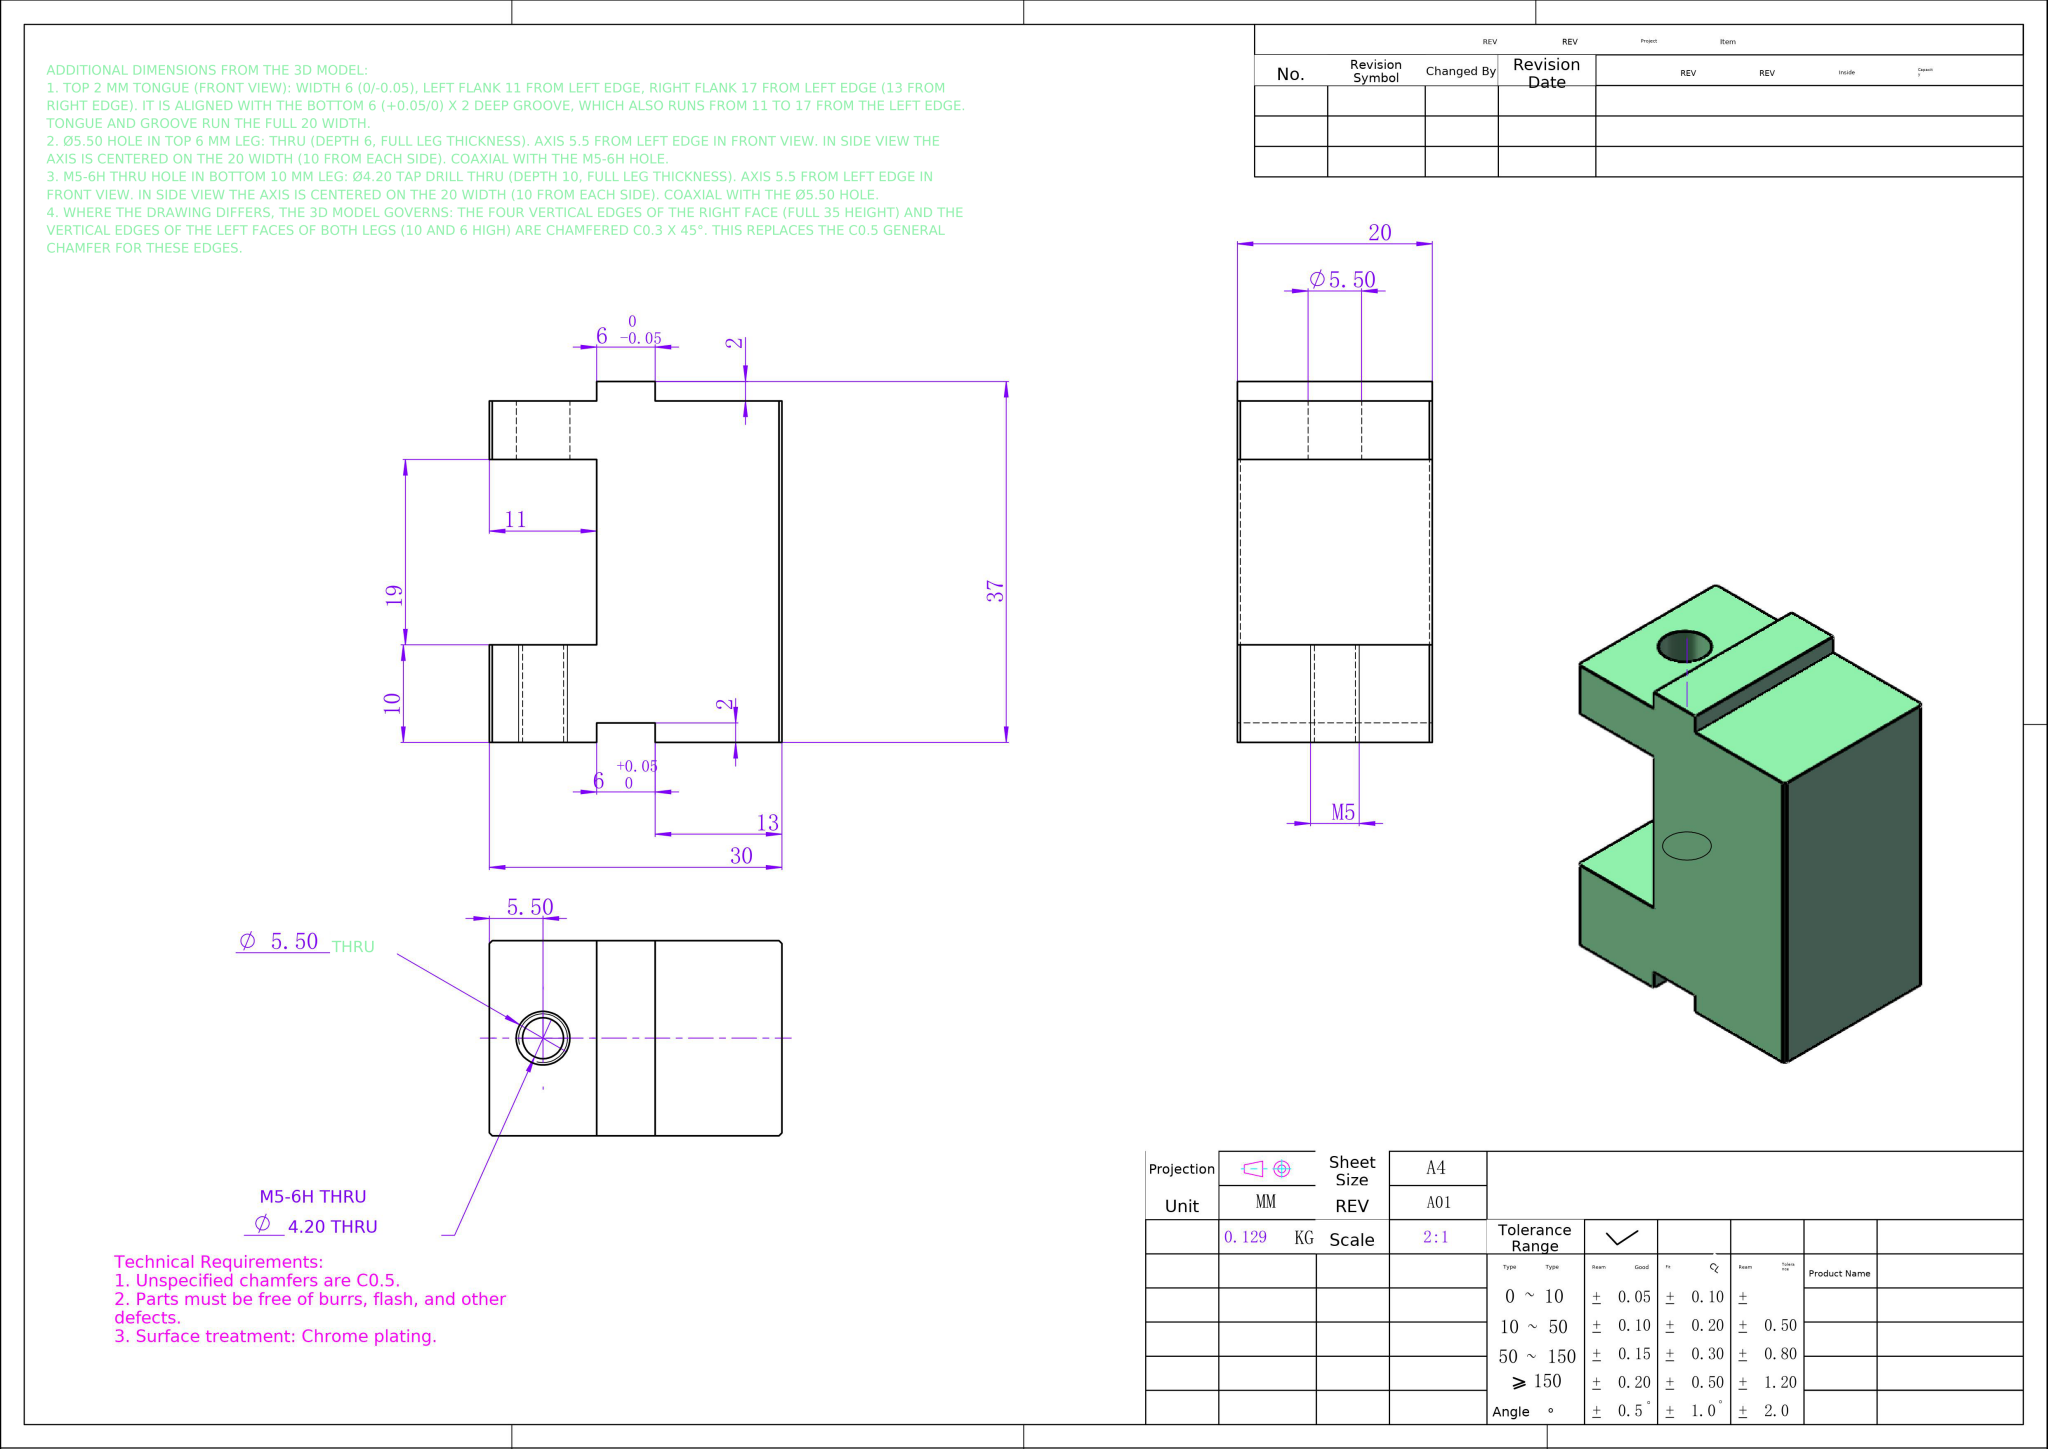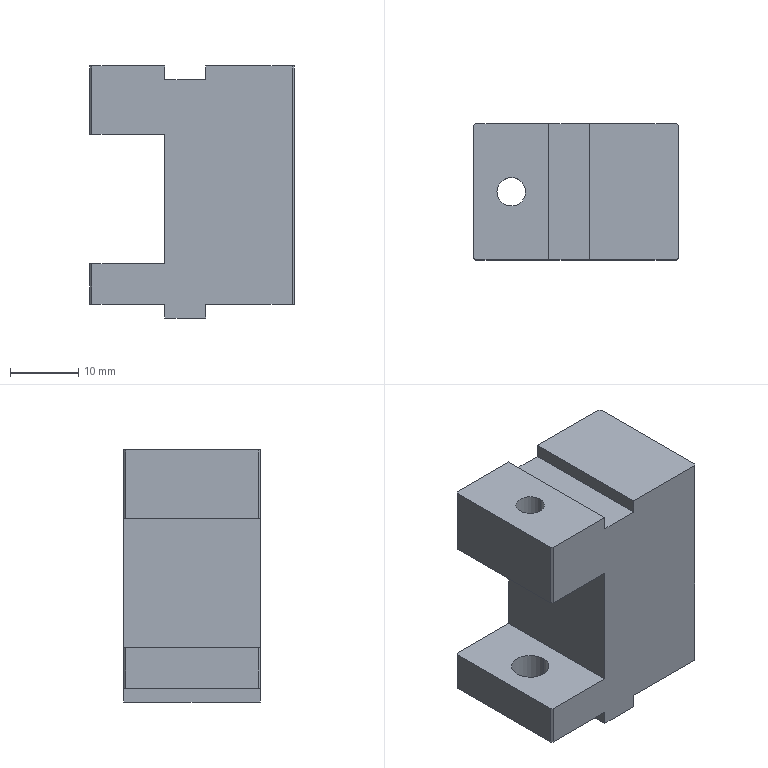Part | NX | mm | 1 solid | 28 faces | box 30 x 20 x 37 mm | volume 16534 mm3 | plane 24 | cylinder 4 | commonest cylinder face diameters 4.2 x2 5.5 x2
STEP:
#1=COLOUR_RGB('',0.5922,1.,0.7098);
#2=FILL_AREA_STYLE_COLOUR('',#1);
#3=FILL_AREA_STYLE('',(#2));
#4=SURFACE_STYLE_FILL_AREA(#3);
#5=SURFACE_SIDE_STYLE('',(#4));
#6=SURFACE_STYLE_USAGE(.BOTH.,#5);
#7=PRESENTATION_STYLE_ASSIGNMENT((#6));
#8=CARTESIAN_POINT('',(-7.4,0.,17.5));
#9=VERTEX_POINT('',#8);
#10=CARTESIAN_POINT('',(-11.6,0.,17.5));
#11=VERTEX_POINT('',#10);
#12=CARTESIAN_POINT('',(-9.5,0.,17.5));
#13=DIRECTION('',(0.,0.,-1.));
#14=DIRECTION('',(-1.,0.,0.));
#15=AXIS2_PLACEMENT_3D('',#12,#13,#14);
#16=CIRCLE('',#15,2.1);
#17=EDGE_CURVE('',#9,#11,#16,.T.);
#18=ORIENTED_EDGE('',*,*,#17,.F.);
#19=CARTESIAN_POINT('',(-7.4,0.,7.5));
#20=VERTEX_POINT('',#19);
#21=CARTESIAN_POINT('',(-7.4,0.,7.5));
#22=DIRECTION('',(0.,0.,-1.));
#23=VECTOR('',#22,1000.);
#24=LINE('',#21,#23);
#25=EDGE_CURVE('',#9,#20,#24,.T.);
#26=ORIENTED_EDGE('',*,*,#25,.T.);
#27=CARTESIAN_POINT('',(-11.6,0.,7.5));
#28=VERTEX_POINT('',#27);
#29=CARTESIAN_POINT('',(-9.5,0.,7.5));
#30=DIRECTION('',(0.,0.,-1.));
#31=DIRECTION('',(-1.,0.,0.));
#32=AXIS2_PLACEMENT_3D('',#29,#30,#31);
#33=CIRCLE('',#32,2.1);
#34=EDGE_CURVE('',#20,#28,#33,.T.);
#35=ORIENTED_EDGE('',*,*,#34,.T.);
#36=CARTESIAN_POINT('',(-11.6,0.,7.5));
#37=DIRECTION('',(0.,0.,-1.));
#38=VECTOR('',#37,1000.);
#39=LINE('',#36,#38);
#40=EDGE_CURVE('',#11,#28,#39,.T.);
#41=ORIENTED_EDGE('',*,*,#40,.F.);
#42=EDGE_LOOP('',(#18,#26,#35,#41));
#43=FACE_OUTER_BOUND('',#42,.T.);
#44=CARTESIAN_POINT('',(-9.5,0.,7.5));
#45=DIRECTION('',(0.,0.,-1.));
#46=DIRECTION('',(-1.,0.,0.));
#47=AXIS2_PLACEMENT_3D('',#44,#45,#46);
#48=CYLINDRICAL_SURFACE('',#47,2.1);
#49=ADVANCED_FACE('',(#43),#48,.F.);
#50=CARTESIAN_POINT('',(-12.25,0.,-11.5));
#51=VERTEX_POINT('',#50);
#52=CARTESIAN_POINT('',(-6.75,0.,-11.5));
#53=VERTEX_POINT('',#52);
#54=CARTESIAN_POINT('',(-9.5,0.,-11.5));
#55=DIRECTION('',(-0.,0.,1.));
#56=DIRECTION('',(-1.,0.,0.));
#57=AXIS2_PLACEMENT_3D('',#54,#55,#56);
#58=CIRCLE('',#57,2.75);
#59=EDGE_CURVE('',#51,#53,#58,.T.);
#60=ORIENTED_EDGE('',*,*,#59,.T.);
#61=CARTESIAN_POINT('',(-6.75,0.,-17.5));
#62=VERTEX_POINT('',#61);
#63=CARTESIAN_POINT('',(-6.75,0.,-17.5));
#64=DIRECTION('',(0.,0.,-1.));
#65=VECTOR('',#64,1000.);
#66=LINE('',#63,#65);
#67=EDGE_CURVE('',#53,#62,#66,.T.);
#68=ORIENTED_EDGE('',*,*,#67,.T.);
#69=CARTESIAN_POINT('',(-12.25,0.,-17.5));
#70=VERTEX_POINT('',#69);
#71=CARTESIAN_POINT('',(-9.5,0.,-17.5));
#72=DIRECTION('',(0.,0.,-1.));
#73=DIRECTION('',(-1.,0.,0.));
#74=AXIS2_PLACEMENT_3D('',#71,#72,#73);
#75=CIRCLE('',#74,2.75);
#76=EDGE_CURVE('',#62,#70,#75,.T.);
#77=ORIENTED_EDGE('',*,*,#76,.T.);
#78=CARTESIAN_POINT('',(-12.25,0.,-17.5));
#79=DIRECTION('',(0.,0.,-1.));
#80=VECTOR('',#79,1000.);
#81=LINE('',#78,#80);
#82=EDGE_CURVE('',#51,#70,#81,.T.);
#83=ORIENTED_EDGE('',*,*,#82,.F.);
#84=EDGE_LOOP('',(#60,#68,#77,#83));
#85=FACE_OUTER_BOUND('',#84,.T.);
#86=CARTESIAN_POINT('',(-9.5,0.,-17.5));
#87=DIRECTION('',(0.,0.,-1.));
#88=DIRECTION('',(-1.,0.,0.));
#89=AXIS2_PLACEMENT_3D('',#86,#87,#88);
#90=CYLINDRICAL_SURFACE('',#89,2.75);
#91=ADVANCED_FACE('',(#85),#90,.F.);
#92=CARTESIAN_POINT('',(-14.7,-10.,7.5));
#93=VERTEX_POINT('',#92);
#94=CARTESIAN_POINT('',(-15.,-9.7,7.5));
#95=VERTEX_POINT('',#94);
#96=CARTESIAN_POINT('',(-14.7,-10.,7.5));
#97=DIRECTION('',(-0.7071,0.7071,-0.));
#98=VECTOR('',#97,1000.);
#99=LINE('',#96,#98);
#100=EDGE_CURVE('',#93,#95,#99,.T.);
#101=ORIENTED_EDGE('',*,*,#100,.T.);
#102=CARTESIAN_POINT('',(-15.,9.7,7.5));
#103=VERTEX_POINT('',#102);
#104=CARTESIAN_POINT('',(-15.,-10.,7.5));
#105=DIRECTION('',(0.,-1.,0.));
#106=VECTOR('',#105,1000.);
#107=LINE('',#104,#106);
#108=EDGE_CURVE('',#103,#95,#107,.T.);
#109=ORIENTED_EDGE('',*,*,#108,.F.);
#110=CARTESIAN_POINT('',(-14.7,10.,7.5));
#111=VERTEX_POINT('',#110);
#112=CARTESIAN_POINT('',(-15.,9.7,7.5));
#113=DIRECTION('',(0.7071,0.7071,0.));
#114=VECTOR('',#113,1000.);
#115=LINE('',#112,#114);
#116=EDGE_CURVE('',#103,#111,#115,.T.);
#117=ORIENTED_EDGE('',*,*,#116,.T.);
#118=CARTESIAN_POINT('',(-4.,10.,7.5));
#119=VERTEX_POINT('',#118);
#120=CARTESIAN_POINT('',(-4.,10.,7.5));
#121=DIRECTION('',(-1.,0.,-0.));
#122=VECTOR('',#121,1000.);
#123=LINE('',#120,#122);
#124=EDGE_CURVE('',#119,#111,#123,.T.);
#125=ORIENTED_EDGE('',*,*,#124,.F.);
#126=CARTESIAN_POINT('',(-4.,-10.,7.5));
#127=VERTEX_POINT('',#126);
#128=CARTESIAN_POINT('',(-4.,10.,7.5));
#129=DIRECTION('',(0.,-1.,0.));
#130=VECTOR('',#129,1000.);
#131=LINE('',#128,#130);
#132=EDGE_CURVE('',#119,#127,#131,.T.);
#133=ORIENTED_EDGE('',*,*,#132,.T.);
#134=CARTESIAN_POINT('',(-4.,-10.,7.5));
#135=DIRECTION('',(-1.,0.,-0.));
#136=VECTOR('',#135,1000.);
#137=LINE('',#134,#136);
#138=EDGE_CURVE('',#127,#93,#137,.T.);
#139=ORIENTED_EDGE('',*,*,#138,.T.);
#140=EDGE_LOOP('',(#101,#109,#117,#125,#133,#139));
#141=FACE_OUTER_BOUND('',#140,.T.);
#142=CARTESIAN_POINT('',(-9.5,0.,7.5));
#143=DIRECTION('',(0.,0.,-1.));
#144=DIRECTION('',(-1.,0.,0.));
#145=AXIS2_PLACEMENT_3D('',#142,#143,#144);
#146=CIRCLE('',#145,2.1);
#147=EDGE_CURVE('',#28,#20,#146,.T.);
#148=ORIENTED_EDGE('',*,*,#147,.F.);
#149=ORIENTED_EDGE('',*,*,#34,.F.);
#150=EDGE_LOOP('',(#148,#149));
#151=FACE_BOUND('',#150,.T.);
#152=CARTESIAN_POINT('',(-4.,10.,7.5));
#153=DIRECTION('',(-0.,0.,1.));
#154=DIRECTION('',(1.,0.,0.));
#155=AXIS2_PLACEMENT_3D('',#152,#153,#154);
#156=PLANE('',#155);
#157=ADVANCED_FACE('',(#141,#151),#156,.F.);
#158=CARTESIAN_POINT('',(-15.,-9.7,-17.5));
#159=VERTEX_POINT('',#158);
#160=CARTESIAN_POINT('',(-15.,-9.7,-11.5));
#161=VERTEX_POINT('',#160);
#162=CARTESIAN_POINT('',(-15.,-9.7,17.5));
#163=DIRECTION('',(0.,0.,1.));
#164=VECTOR('',#163,1000.);
#165=LINE('',#162,#164);
#166=EDGE_CURVE('',#159,#161,#165,.T.);
#167=ORIENTED_EDGE('',*,*,#166,.T.);
#168=CARTESIAN_POINT('',(-15.,9.7,-11.5));
#169=VERTEX_POINT('',#168);
#170=CARTESIAN_POINT('',(-15.,-10.,-11.5));
#171=DIRECTION('',(0.,1.,0.));
#172=VECTOR('',#171,1000.);
#173=LINE('',#170,#172);
#174=EDGE_CURVE('',#161,#169,#173,.T.);
#175=ORIENTED_EDGE('',*,*,#174,.T.);
#176=CARTESIAN_POINT('',(-15.,9.7,-17.5));
#177=VERTEX_POINT('',#176);
#178=CARTESIAN_POINT('',(-15.,9.7,17.5));
#179=DIRECTION('',(0.,0.,-1.));
#180=VECTOR('',#179,1000.);
#181=LINE('',#178,#180);
#182=EDGE_CURVE('',#169,#177,#181,.T.);
#183=ORIENTED_EDGE('',*,*,#182,.T.);
#184=CARTESIAN_POINT('',(-15.,-10.,-17.5));
#185=DIRECTION('',(0.,-1.,0.));
#186=VECTOR('',#185,1000.);
#187=LINE('',#184,#186);
#188=EDGE_CURVE('',#177,#159,#187,.T.);
#189=ORIENTED_EDGE('',*,*,#188,.T.);
#190=EDGE_LOOP('',(#167,#175,#183,#189));
#191=FACE_OUTER_BOUND('',#190,.T.);
#192=CARTESIAN_POINT('',(-15.,-10.,17.5));
#193=DIRECTION('',(1.,0.,0.));
#194=DIRECTION('',(0.,0.,-1.));
#195=AXIS2_PLACEMENT_3D('',#192,#193,#194);
#196=PLANE('',#195);
#197=ADVANCED_FACE('',(#191),#196,.F.);
#198=CARTESIAN_POINT('',(-14.7,-10.,-11.5));
#199=VERTEX_POINT('',#198);
#200=CARTESIAN_POINT('',(-14.7,-10.,-11.5));
#201=DIRECTION('',(0.7071,-0.7071,0.));
#202=VECTOR('',#201,1000.);
#203=LINE('',#200,#202);
#204=EDGE_CURVE('',#161,#199,#203,.T.);
#205=ORIENTED_EDGE('',*,*,#204,.F.);
#206=ORIENTED_EDGE('',*,*,#166,.F.);
#207=CARTESIAN_POINT('',(-14.7,-10.,-17.5));
#208=VERTEX_POINT('',#207);
#209=CARTESIAN_POINT('',(-12.35,-12.35,-17.5));
#210=DIRECTION('',(-0.7071,0.7071,0.));
#211=VECTOR('',#210,1000.);
#212=LINE('',#209,#211);
#213=EDGE_CURVE('',#208,#159,#212,.T.);
#214=ORIENTED_EDGE('',*,*,#213,.F.);
#215=CARTESIAN_POINT('',(-14.7,-10.,17.5));
#216=DIRECTION('',(0.,0.,-1.));
#217=VECTOR('',#216,1000.);
#218=LINE('',#215,#217);
#219=EDGE_CURVE('',#199,#208,#218,.T.);
#220=ORIENTED_EDGE('',*,*,#219,.F.);
#221=EDGE_LOOP('',(#205,#206,#214,#220));
#222=FACE_OUTER_BOUND('',#221,.T.);
#223=CARTESIAN_POINT('',(-14.7,-10.,17.5));
#224=DIRECTION('',(0.7071,0.7071,0.));
#225=DIRECTION('',(0.,0.,-1.));
#226=AXIS2_PLACEMENT_3D('',#223,#224,#225);
#227=PLANE('',#226);
#228=ADVANCED_FACE('',(#222),#227,.F.);
#229=CARTESIAN_POINT('',(-14.7,10.,-11.5));
#230=VERTEX_POINT('',#229);
#231=CARTESIAN_POINT('',(-15.,9.7,-11.5));
#232=DIRECTION('',(-0.7071,-0.7071,-0.));
#233=VECTOR('',#232,1000.);
#234=LINE('',#231,#233);
#235=EDGE_CURVE('',#230,#169,#234,.T.);
#236=ORIENTED_EDGE('',*,*,#235,.F.);
#237=CARTESIAN_POINT('',(-14.7,10.,-17.5));
#238=VERTEX_POINT('',#237);
#239=CARTESIAN_POINT('',(-14.7,10.,17.5));
#240=DIRECTION('',(0.,0.,1.));
#241=VECTOR('',#240,1000.);
#242=LINE('',#239,#241);
#243=EDGE_CURVE('',#238,#230,#242,.T.);
#244=ORIENTED_EDGE('',*,*,#243,.F.);
#245=CARTESIAN_POINT('',(-12.35,12.35,-17.5));
#246=DIRECTION('',(0.7071,0.7071,0.));
#247=VECTOR('',#246,1000.);
#248=LINE('',#245,#247);
#249=EDGE_CURVE('',#177,#238,#248,.T.);
#250=ORIENTED_EDGE('',*,*,#249,.F.);
#251=ORIENTED_EDGE('',*,*,#182,.F.);
#252=EDGE_LOOP('',(#236,#244,#250,#251));
#253=FACE_OUTER_BOUND('',#252,.T.);
#254=CARTESIAN_POINT('',(-15.,9.7,17.5));
#255=DIRECTION('',(0.7071,-0.7071,0.));
#256=DIRECTION('',(0.,0.,-1.));
#257=AXIS2_PLACEMENT_3D('',#254,#255,#256);
#258=PLANE('',#257);
#259=ADVANCED_FACE('',(#253),#258,.F.);
#260=CARTESIAN_POINT('',(14.7,10.,17.5));
#261=VERTEX_POINT('',#260);
#262=CARTESIAN_POINT('',(2.,10.,17.5));
#263=VERTEX_POINT('',#262);
#264=CARTESIAN_POINT('',(-15.,10.,17.5));
#265=DIRECTION('',(-1.,0.,0.));
#266=VECTOR('',#265,1000.);
#267=LINE('',#264,#266);
#268=EDGE_CURVE('',#261,#263,#267,.T.);
#269=ORIENTED_EDGE('',*,*,#268,.T.);
#270=CARTESIAN_POINT('',(2.,-10.,17.5));
#271=VERTEX_POINT('',#270);
#272=CARTESIAN_POINT('',(2.,10.,17.5));
#273=DIRECTION('',(0.,-1.,0.));
#274=VECTOR('',#273,1000.);
#275=LINE('',#272,#274);
#276=EDGE_CURVE('',#263,#271,#275,.T.);
#277=ORIENTED_EDGE('',*,*,#276,.T.);
#278=CARTESIAN_POINT('',(14.7,-10.,17.5));
#279=VERTEX_POINT('',#278);
#280=CARTESIAN_POINT('',(-15.,-10.,17.5));
#281=DIRECTION('',(1.,0.,0.));
#282=VECTOR('',#281,1000.);
#283=LINE('',#280,#282);
#284=EDGE_CURVE('',#271,#279,#283,.T.);
#285=ORIENTED_EDGE('',*,*,#284,.T.);
#286=CARTESIAN_POINT('',(15.,-9.7,17.5));
#287=VERTEX_POINT('',#286);
#288=CARTESIAN_POINT('',(15.,-9.7,17.5));
#289=DIRECTION('',(0.7071,0.7071,0.));
#290=VECTOR('',#289,1000.);
#291=LINE('',#288,#290);
#292=EDGE_CURVE('',#279,#287,#291,.T.);
#293=ORIENTED_EDGE('',*,*,#292,.T.);
#294=CARTESIAN_POINT('',(15.,9.7,17.5));
#295=VERTEX_POINT('',#294);
#296=CARTESIAN_POINT('',(15.,-10.,17.5));
#297=DIRECTION('',(0.,1.,0.));
#298=VECTOR('',#297,1000.);
#299=LINE('',#296,#298);
#300=EDGE_CURVE('',#287,#295,#299,.T.);
#301=ORIENTED_EDGE('',*,*,#300,.T.);
#302=CARTESIAN_POINT('',(14.7,10.,17.5));
#303=DIRECTION('',(-0.7071,0.7071,0.));
#304=VECTOR('',#303,1000.);
#305=LINE('',#302,#304);
#306=EDGE_CURVE('',#295,#261,#305,.T.);
#307=ORIENTED_EDGE('',*,*,#306,.T.);
#308=EDGE_LOOP('',(#269,#277,#285,#293,#301,#307));
#309=FACE_OUTER_BOUND('',#308,.T.);
#310=CARTESIAN_POINT('',(0.,0.,17.5));
#311=DIRECTION('',(0.,0.,-1.));
#312=DIRECTION('',(-1.,0.,0.));
#313=AXIS2_PLACEMENT_3D('',#310,#311,#312);
#314=PLANE('',#313);
#315=ADVANCED_FACE('',(#309),#314,.F.);
#316=CARTESIAN_POINT('',(-9.5,0.,-17.5));
#317=DIRECTION('',(0.,0.,-1.));
#318=DIRECTION('',(-1.,0.,0.));
#319=AXIS2_PLACEMENT_3D('',#316,#317,#318);
#320=CIRCLE('',#319,2.75);
#321=EDGE_CURVE('',#70,#62,#320,.T.);
#322=ORIENTED_EDGE('',*,*,#321,.F.);
#323=ORIENTED_EDGE('',*,*,#76,.F.);
#324=EDGE_LOOP('',(#322,#323));
#325=FACE_BOUND('',#324,.T.);
#326=CARTESIAN_POINT('',(-4.,-10.,-17.5));
#327=VERTEX_POINT('',#326);
#328=CARTESIAN_POINT('',(-4.,10.,-17.5));
#329=VERTEX_POINT('',#328);
#330=CARTESIAN_POINT('',(-4.,10.,-17.5));
#331=DIRECTION('',(0.,1.,0.));
#332=VECTOR('',#331,1000.);
#333=LINE('',#330,#332);
#334=EDGE_CURVE('',#327,#329,#333,.T.);
#335=ORIENTED_EDGE('',*,*,#334,.F.);
#336=CARTESIAN_POINT('',(-15.,-10.,-17.5));
#337=DIRECTION('',(1.,0.,0.));
#338=VECTOR('',#337,1000.);
#339=LINE('',#336,#338);
#340=EDGE_CURVE('',#208,#327,#339,.T.);
#341=ORIENTED_EDGE('',*,*,#340,.F.);
#342=ORIENTED_EDGE('',*,*,#213,.T.);
#343=ORIENTED_EDGE('',*,*,#188,.F.);
#344=ORIENTED_EDGE('',*,*,#249,.T.);
#345=CARTESIAN_POINT('',(-15.,10.,-17.5));
#346=DIRECTION('',(-1.,0.,0.));
#347=VECTOR('',#346,1000.);
#348=LINE('',#345,#347);
#349=EDGE_CURVE('',#329,#238,#348,.T.);
#350=ORIENTED_EDGE('',*,*,#349,.F.);
#351=EDGE_LOOP('',(#335,#341,#342,#343,#344,#350));
#352=FACE_OUTER_BOUND('',#351,.T.);
#353=CARTESIAN_POINT('',(0.,0.,-17.5));
#354=DIRECTION('',(0.,0.,-1.));
#355=DIRECTION('',(-1.,0.,0.));
#356=AXIS2_PLACEMENT_3D('',#353,#354,#355);
#357=PLANE('',#356);
#358=ADVANCED_FACE('',(#325,#352),#357,.T.);
#359=ORIENTED_EDGE('',*,*,#300,.F.);
#360=CARTESIAN_POINT('',(15.,-9.7,-17.5));
#361=VERTEX_POINT('',#360);
#362=CARTESIAN_POINT('',(15.,-9.7,17.5));
#363=DIRECTION('',(0.,0.,-1.));
#364=VECTOR('',#363,1000.);
#365=LINE('',#362,#364);
#366=EDGE_CURVE('',#287,#361,#365,.T.);
#367=ORIENTED_EDGE('',*,*,#366,.T.);
#368=CARTESIAN_POINT('',(15.,9.7,-17.5));
#369=VERTEX_POINT('',#368);
#370=CARTESIAN_POINT('',(15.,-10.,-17.5));
#371=DIRECTION('',(0.,1.,0.));
#372=VECTOR('',#371,1000.);
#373=LINE('',#370,#372);
#374=EDGE_CURVE('',#361,#369,#373,.T.);
#375=ORIENTED_EDGE('',*,*,#374,.T.);
#376=CARTESIAN_POINT('',(15.,9.7,17.5));
#377=DIRECTION('',(0.,0.,1.));
#378=VECTOR('',#377,1000.);
#379=LINE('',#376,#378);
#380=EDGE_CURVE('',#369,#295,#379,.T.);
#381=ORIENTED_EDGE('',*,*,#380,.T.);
#382=EDGE_LOOP('',(#359,#367,#375,#381));
#383=FACE_OUTER_BOUND('',#382,.T.);
#384=CARTESIAN_POINT('',(15.,-10.,17.5));
#385=DIRECTION('',(-1.,0.,0.));
#386=DIRECTION('',(0.,0.,1.));
#387=AXIS2_PLACEMENT_3D('',#384,#385,#386);
#388=PLANE('',#387);
#389=ADVANCED_FACE('',(#383),#388,.F.);
#390=ORIENTED_EDGE('',*,*,#243,.T.);
#391=CARTESIAN_POINT('',(-4.,10.,-11.5));
#392=VERTEX_POINT('',#391);
#393=CARTESIAN_POINT('',(-4.,10.,-11.5));
#394=DIRECTION('',(1.,0.,0.));
#395=VECTOR('',#394,1000.);
#396=LINE('',#393,#395);
#397=EDGE_CURVE('',#230,#392,#396,.T.);
#398=ORIENTED_EDGE('',*,*,#397,.T.);
#399=CARTESIAN_POINT('',(-4.,10.,-11.5));
#400=DIRECTION('',(0.,0.,1.));
#401=VECTOR('',#400,1000.);
#402=LINE('',#399,#401);
#403=EDGE_CURVE('',#392,#119,#402,.T.);
#404=ORIENTED_EDGE('',*,*,#403,.T.);
#405=ORIENTED_EDGE('',*,*,#124,.T.);
#406=CARTESIAN_POINT('',(-14.7,10.,17.5));
#407=VERTEX_POINT('',#406);
#408=CARTESIAN_POINT('',(-14.7,10.,17.5));
#409=DIRECTION('',(0.,0.,1.));
#410=VECTOR('',#409,1000.);
#411=LINE('',#408,#410);
#412=EDGE_CURVE('',#111,#407,#411,.T.);
#413=ORIENTED_EDGE('',*,*,#412,.T.);
#414=CARTESIAN_POINT('',(-4.,10.,17.5));
#415=VERTEX_POINT('',#414);
#416=CARTESIAN_POINT('',(-15.,10.,17.5));
#417=DIRECTION('',(-1.,0.,0.));
#418=VECTOR('',#417,1000.);
#419=LINE('',#416,#418);
#420=EDGE_CURVE('',#415,#407,#419,.T.);
#421=ORIENTED_EDGE('',*,*,#420,.F.);
#422=CARTESIAN_POINT('',(-4.,10.,15.5));
#423=VERTEX_POINT('',#422);
#424=CARTESIAN_POINT('',(-4.,10.,17.5));
#425=DIRECTION('',(0.,0.,-1.));
#426=VECTOR('',#425,1000.);
#427=LINE('',#424,#426);
#428=EDGE_CURVE('',#415,#423,#427,.T.);
#429=ORIENTED_EDGE('',*,*,#428,.T.);
#430=CARTESIAN_POINT('',(2.,10.,15.5));
#431=VERTEX_POINT('',#430);
#432=CARTESIAN_POINT('',(2.,10.,15.5));
#433=DIRECTION('',(1.,0.,0.));
#434=VECTOR('',#433,1000.);
#435=LINE('',#432,#434);
#436=EDGE_CURVE('',#423,#431,#435,.T.);
#437=ORIENTED_EDGE('',*,*,#436,.T.);
#438=CARTESIAN_POINT('',(2.,10.,17.5));
#439=DIRECTION('',(-0.,0.,1.));
#440=VECTOR('',#439,1000.);
#441=LINE('',#438,#440);
#442=EDGE_CURVE('',#431,#263,#441,.T.);
#443=ORIENTED_EDGE('',*,*,#442,.T.);
#444=ORIENTED_EDGE('',*,*,#268,.F.);
#445=CARTESIAN_POINT('',(14.7,10.,-17.5));
#446=VERTEX_POINT('',#445);
#447=CARTESIAN_POINT('',(14.7,10.,17.5));
#448=DIRECTION('',(0.,0.,-1.));
#449=VECTOR('',#448,1000.);
#450=LINE('',#447,#449);
#451=EDGE_CURVE('',#261,#446,#450,.T.);
#452=ORIENTED_EDGE('',*,*,#451,.T.);
#453=CARTESIAN_POINT('',(2.,10.,-17.5));
#454=VERTEX_POINT('',#453);
#455=CARTESIAN_POINT('',(-15.,10.,-17.5));
#456=DIRECTION('',(-1.,0.,0.));
#457=VECTOR('',#456,1000.);
#458=LINE('',#455,#457);
#459=EDGE_CURVE('',#446,#454,#458,.T.);
#460=ORIENTED_EDGE('',*,*,#459,.T.);
#461=CARTESIAN_POINT('',(2.,10.,-19.5));
#462=VERTEX_POINT('',#461);
#463=CARTESIAN_POINT('',(2.,10.,-19.5));
#464=DIRECTION('',(0.,0.,1.));
#465=VECTOR('',#464,1000.);
#466=LINE('',#463,#465);
#467=EDGE_CURVE('',#462,#454,#466,.T.);
#468=ORIENTED_EDGE('',*,*,#467,.F.);
#469=CARTESIAN_POINT('',(-4.,10.,-19.5));
#470=VERTEX_POINT('',#469);
#471=CARTESIAN_POINT('',(2.,10.,-19.5));
#472=DIRECTION('',(1.,0.,0.));
#473=VECTOR('',#472,1000.);
#474=LINE('',#471,#473);
#475=EDGE_CURVE('',#470,#462,#474,.T.);
#476=ORIENTED_EDGE('',*,*,#475,.F.);
#477=CARTESIAN_POINT('',(-4.,10.,-19.5));
#478=DIRECTION('',(0.,0.,1.));
#479=VECTOR('',#478,1000.);
#480=LINE('',#477,#479);
#481=EDGE_CURVE('',#470,#329,#480,.T.);
#482=ORIENTED_EDGE('',*,*,#481,.T.);
#483=ORIENTED_EDGE('',*,*,#349,.T.);
#484=EDGE_LOOP('',(#390,#398,#404,#405,#413,#421,#429,#437,#443,#444,#452,#460,#468,#476,#482,#483));
#485=FACE_OUTER_BOUND('',#484,.T.);
#486=CARTESIAN_POINT('',(-15.,10.,17.5));
#487=DIRECTION('',(0.,-1.,0.));
#488=DIRECTION('',(0.,0.,-1.));
#489=AXIS2_PLACEMENT_3D('',#486,#487,#488);
#490=PLANE('',#489);
#491=ADVANCED_FACE('',(#485),#490,.F.);
#492=CARTESIAN_POINT('',(-15.,9.7,17.5));
#493=VERTEX_POINT('',#492);
#494=CARTESIAN_POINT('',(-15.,9.7,17.5));
#495=DIRECTION('',(0.,0.,-1.));
#496=VECTOR('',#495,1000.);
#497=LINE('',#494,#496);
#498=EDGE_CURVE('',#493,#103,#497,.T.);
#499=ORIENTED_EDGE('',*,*,#498,.T.);
#500=ORIENTED_EDGE('',*,*,#108,.T.);
#501=CARTESIAN_POINT('',(-15.,-9.7,17.5));
#502=VERTEX_POINT('',#501);
#503=CARTESIAN_POINT('',(-15.,-9.7,17.5));
#504=DIRECTION('',(0.,0.,1.));
#505=VECTOR('',#504,1000.);
#506=LINE('',#503,#505);
#507=EDGE_CURVE('',#95,#502,#506,.T.);
#508=ORIENTED_EDGE('',*,*,#507,.T.);
#509=CARTESIAN_POINT('',(-15.,-10.,17.5));
#510=DIRECTION('',(0.,-1.,0.));
#511=VECTOR('',#510,1000.);
#512=LINE('',#509,#511);
#513=EDGE_CURVE('',#493,#502,#512,.T.);
#514=ORIENTED_EDGE('',*,*,#513,.F.);
#515=EDGE_LOOP('',(#499,#500,#508,#514));
#516=FACE_OUTER_BOUND('',#515,.T.);
#517=CARTESIAN_POINT('',(-15.,-10.,17.5));
#518=DIRECTION('',(1.,0.,0.));
#519=DIRECTION('',(0.,0.,-1.));
#520=AXIS2_PLACEMENT_3D('',#517,#518,#519);
#521=PLANE('',#520);
#522=ADVANCED_FACE('',(#516),#521,.F.);
#523=CARTESIAN_POINT('',(-4.,-10.,-11.5));
#524=VERTEX_POINT('',#523);
#525=CARTESIAN_POINT('',(-4.,-10.,-11.5));
#526=DIRECTION('',(0.,0.,1.));
#527=VECTOR('',#526,1000.);
#528=LINE('',#525,#527);
#529=EDGE_CURVE('',#524,#127,#528,.T.);
#530=ORIENTED_EDGE('',*,*,#529,.F.);
#531=CARTESIAN_POINT('',(-4.,-10.,-11.5));
#532=DIRECTION('',(1.,0.,0.));
#533=VECTOR('',#532,1000.);
#534=LINE('',#531,#533);
#535=EDGE_CURVE('',#199,#524,#534,.T.);
#536=ORIENTED_EDGE('',*,*,#535,.F.);
#537=ORIENTED_EDGE('',*,*,#219,.T.);
#538=ORIENTED_EDGE('',*,*,#340,.T.);
#539=CARTESIAN_POINT('',(-4.,-10.,-19.5));
#540=VERTEX_POINT('',#539);
#541=CARTESIAN_POINT('',(-4.,-10.,-19.5));
#542=DIRECTION('',(0.,0.,1.));
#543=VECTOR('',#542,1000.);
#544=LINE('',#541,#543);
#545=EDGE_CURVE('',#540,#327,#544,.T.);
#546=ORIENTED_EDGE('',*,*,#545,.F.);
#547=CARTESIAN_POINT('',(2.,-10.,-19.5));
#548=VERTEX_POINT('',#547);
#549=CARTESIAN_POINT('',(2.,-10.,-19.5));
#550=DIRECTION('',(-1.,0.,0.));
#551=VECTOR('',#550,1000.);
#552=LINE('',#549,#551);
#553=EDGE_CURVE('',#548,#540,#552,.T.);
#554=ORIENTED_EDGE('',*,*,#553,.F.);
#555=CARTESIAN_POINT('',(2.,-10.,-17.5));
#556=VERTEX_POINT('',#555);
#557=CARTESIAN_POINT('',(2.,-10.,-19.5));
#558=DIRECTION('',(0.,0.,1.));
#559=VECTOR('',#558,1000.);
#560=LINE('',#557,#559);
#561=EDGE_CURVE('',#548,#556,#560,.T.);
#562=ORIENTED_EDGE('',*,*,#561,.T.);
#563=CARTESIAN_POINT('',(14.7,-10.,-17.5));
#564=VERTEX_POINT('',#563);
#565=CARTESIAN_POINT('',(-15.,-10.,-17.5));
#566=DIRECTION('',(1.,0.,0.));
#567=VECTOR('',#566,1000.);
#568=LINE('',#565,#567);
#569=EDGE_CURVE('',#556,#564,#568,.T.);
#570=ORIENTED_EDGE('',*,*,#569,.T.);
#571=CARTESIAN_POINT('',(14.7,-10.,17.5));
#572=DIRECTION('',(0.,0.,1.));
#573=VECTOR('',#572,1000.);
#574=LINE('',#571,#573);
#575=EDGE_CURVE('',#564,#279,#574,.T.);
#576=ORIENTED_EDGE('',*,*,#575,.T.);
#577=ORIENTED_EDGE('',*,*,#284,.F.);
#578=CARTESIAN_POINT('',(2.,-10.,15.5));
#579=VERTEX_POINT('',#578);
#580=CARTESIAN_POINT('',(2.,-10.,17.5));
#581=DIRECTION('',(-0.,0.,1.));
#582=VECTOR('',#581,1000.);
#583=LINE('',#580,#582);
#584=EDGE_CURVE('',#579,#271,#583,.T.);
#585=ORIENTED_EDGE('',*,*,#584,.F.);
#586=CARTESIAN_POINT('',(-4.,-10.,15.5));
#587=VERTEX_POINT('',#586);
#588=CARTESIAN_POINT('',(2.,-10.,15.5));
#589=DIRECTION('',(1.,0.,0.));
#590=VECTOR('',#589,1000.);
#591=LINE('',#588,#590);
#592=EDGE_CURVE('',#587,#579,#591,.T.);
#593=ORIENTED_EDGE('',*,*,#592,.F.);
#594=CARTESIAN_POINT('',(-4.,-10.,17.5));
#595=VERTEX_POINT('',#594);
#596=CARTESIAN_POINT('',(-4.,-10.,17.5));
#597=DIRECTION('',(0.,0.,-1.));
#598=VECTOR('',#597,1000.);
#599=LINE('',#596,#598);
#600=EDGE_CURVE('',#595,#587,#599,.T.);
#601=ORIENTED_EDGE('',*,*,#600,.F.);
#602=CARTESIAN_POINT('',(-14.7,-10.,17.5));
#603=VERTEX_POINT('',#602);
#604=CARTESIAN_POINT('',(-15.,-10.,17.5));
#605=DIRECTION('',(1.,0.,0.));
#606=VECTOR('',#605,1000.);
#607=LINE('',#604,#606);
#608=EDGE_CURVE('',#603,#595,#607,.T.);
#609=ORIENTED_EDGE('',*,*,#608,.F.);
#610=CARTESIAN_POINT('',(-14.7,-10.,17.5));
#611=DIRECTION('',(0.,0.,-1.));
#612=VECTOR('',#611,1000.);
#613=LINE('',#610,#612);
#614=EDGE_CURVE('',#603,#93,#613,.T.);
#615=ORIENTED_EDGE('',*,*,#614,.T.);
#616=ORIENTED_EDGE('',*,*,#138,.F.);
#617=EDGE_LOOP('',(#530,#536,#537,#538,#546,#554,#562,#570,#576,#577,#585,#593,#601,#609,#615,#616));
#618=FACE_OUTER_BOUND('',#617,.T.);
#619=CARTESIAN_POINT('',(-15.,-10.,17.5));
#620=DIRECTION('',(0.,1.,0.));
#621=DIRECTION('',(0.,0.,1.));
#622=AXIS2_PLACEMENT_3D('',#619,#620,#621);
#623=PLANE('',#622);
#624=ADVANCED_FACE('',(#618),#623,.F.);
#625=CARTESIAN_POINT('',(-9.5,0.,17.5));
#626=DIRECTION('',(0.,0.,-1.));
#627=DIRECTION('',(-1.,0.,0.));
#628=AXIS2_PLACEMENT_3D('',#625,#626,#627);
#629=CIRCLE('',#628,2.1);
#630=EDGE_CURVE('',#11,#9,#629,.T.);
#631=ORIENTED_EDGE('',*,*,#630,.T.);
#632=ORIENTED_EDGE('',*,*,#17,.T.);
#633=EDGE_LOOP('',(#631,#632));
#634=FACE_BOUND('',#633,.T.);
#635=ORIENTED_EDGE('',*,*,#608,.T.);
#636=CARTESIAN_POINT('',(-4.,10.,17.5));
#637=DIRECTION('',(0.,-1.,0.));
#638=VECTOR('',#637,1000.);
#639=LINE('',#636,#638);
#640=EDGE_CURVE('',#415,#595,#639,.T.);
#641=ORIENTED_EDGE('',*,*,#640,.F.);
#642=ORIENTED_EDGE('',*,*,#420,.T.);
#643=CARTESIAN_POINT('',(-15.,9.7,17.5));
#644=DIRECTION('',(-0.7071,-0.7071,0.));
#645=VECTOR('',#644,1000.);
#646=LINE('',#643,#645);
#647=EDGE_CURVE('',#407,#493,#646,.T.);
#648=ORIENTED_EDGE('',*,*,#647,.T.);
#649=ORIENTED_EDGE('',*,*,#513,.T.);
#650=CARTESIAN_POINT('',(-14.7,-10.,17.5));
#651=DIRECTION('',(0.7071,-0.7071,0.));
#652=VECTOR('',#651,1000.);
#653=LINE('',#650,#652);
#654=EDGE_CURVE('',#502,#603,#653,.T.);
#655=ORIENTED_EDGE('',*,*,#654,.T.);
#656=EDGE_LOOP('',(#635,#641,#642,#648,#649,#655));
#657=FACE_OUTER_BOUND('',#656,.T.);
#658=CARTESIAN_POINT('',(0.,0.,17.5));
#659=DIRECTION('',(0.,0.,-1.));
#660=DIRECTION('',(-1.,0.,0.));
#661=AXIS2_PLACEMENT_3D('',#658,#659,#660);
#662=PLANE('',#661);
#663=ADVANCED_FACE('',(#634,#657),#662,.F.);
#664=CARTESIAN_POINT('',(2.,10.,-17.5));
#665=DIRECTION('',(-0.,-1.,0.));
#666=VECTOR('',#665,1000.);
#667=LINE('',#664,#666);
#668=EDGE_CURVE('',#454,#556,#667,.T.);
#669=ORIENTED_EDGE('',*,*,#668,.F.);
#670=ORIENTED_EDGE('',*,*,#459,.F.);
#671=CARTESIAN_POINT('',(12.35,12.35,-17.5));
#672=DIRECTION('',(0.7071,-0.7071,0.));
#673=VECTOR('',#672,1000.);
#674=LINE('',#671,#673);
#675=EDGE_CURVE('',#446,#369,#674,.T.);
#676=ORIENTED_EDGE('',*,*,#675,.T.);
#677=ORIENTED_EDGE('',*,*,#374,.F.);
#678=CARTESIAN_POINT('',(12.35,-12.35,-17.5));
#679=DIRECTION('',(-0.7071,-0.7071,0.));
#680=VECTOR('',#679,1000.);
#681=LINE('',#678,#680);
#682=EDGE_CURVE('',#361,#564,#681,.T.);
#683=ORIENTED_EDGE('',*,*,#682,.T.);
#684=ORIENTED_EDGE('',*,*,#569,.F.);
#685=EDGE_LOOP('',(#669,#670,#676,#677,#683,#684));
#686=FACE_OUTER_BOUND('',#685,.T.);
#687=CARTESIAN_POINT('',(0.,0.,-17.5));
#688=DIRECTION('',(0.,0.,-1.));
#689=DIRECTION('',(-1.,0.,0.));
#690=AXIS2_PLACEMENT_3D('',#687,#688,#689);
#691=PLANE('',#690);
#692=ADVANCED_FACE('',(#686),#691,.T.);
#693=ORIENTED_EDGE('',*,*,#100,.F.);
#694=ORIENTED_EDGE('',*,*,#614,.F.);
#695=ORIENTED_EDGE('',*,*,#654,.F.);
#696=ORIENTED_EDGE('',*,*,#507,.F.);
#697=EDGE_LOOP('',(#693,#694,#695,#696));
#698=FACE_OUTER_BOUND('',#697,.T.);
#699=CARTESIAN_POINT('',(-14.7,-10.,17.5));
#700=DIRECTION('',(0.7071,0.7071,0.));
#701=DIRECTION('',(0.,0.,-1.));
#702=AXIS2_PLACEMENT_3D('',#699,#700,#701);
#703=PLANE('',#702);
#704=ADVANCED_FACE('',(#698),#703,.F.);
#705=ORIENTED_EDGE('',*,*,#116,.F.);
#706=ORIENTED_EDGE('',*,*,#498,.F.);
#707=ORIENTED_EDGE('',*,*,#647,.F.);
#708=ORIENTED_EDGE('',*,*,#412,.F.);
#709=EDGE_LOOP('',(#705,#706,#707,#708));
#710=FACE_OUTER_BOUND('',#709,.T.);
#711=CARTESIAN_POINT('',(-15.,9.7,17.5));
#712=DIRECTION('',(0.7071,-0.7071,0.));
#713=DIRECTION('',(0.,0.,-1.));
#714=AXIS2_PLACEMENT_3D('',#711,#712,#713);
#715=PLANE('',#714);
#716=ADVANCED_FACE('',(#710),#715,.F.);
#717=ORIENTED_EDGE('',*,*,#292,.F.);
#718=ORIENTED_EDGE('',*,*,#575,.F.);
#719=ORIENTED_EDGE('',*,*,#682,.F.);
#720=ORIENTED_EDGE('',*,*,#366,.F.);
#721=EDGE_LOOP('',(#717,#718,#719,#720));
#722=FACE_OUTER_BOUND('',#721,.T.);
#723=CARTESIAN_POINT('',(15.,-9.7,17.5));
#724=DIRECTION('',(-0.7071,0.7071,0.));
#725=DIRECTION('',(0.,0.,-1.));
#726=AXIS2_PLACEMENT_3D('',#723,#724,#725);
#727=PLANE('',#726);
#728=ADVANCED_FACE('',(#722),#727,.F.);
#729=ORIENTED_EDGE('',*,*,#306,.F.);
#730=ORIENTED_EDGE('',*,*,#380,.F.);
#731=ORIENTED_EDGE('',*,*,#675,.F.);
#732=ORIENTED_EDGE('',*,*,#451,.F.);
#733=EDGE_LOOP('',(#729,#730,#731,#732));
#734=FACE_OUTER_BOUND('',#733,.T.);
#735=CARTESIAN_POINT('',(14.7,10.,17.5));
#736=DIRECTION('',(-0.7071,-0.7071,0.));
#737=DIRECTION('',(0.,0.,-1.));
#738=AXIS2_PLACEMENT_3D('',#735,#736,#737);
#739=PLANE('',#738);
#740=ADVANCED_FACE('',(#734),#739,.F.);
#741=ORIENTED_EDGE('',*,*,#334,.T.);
#742=ORIENTED_EDGE('',*,*,#481,.F.);
#743=CARTESIAN_POINT('',(-4.,10.,-19.5));
#744=DIRECTION('',(0.,1.,0.));
#745=VECTOR('',#744,1000.);
#746=LINE('',#743,#745);
#747=EDGE_CURVE('',#540,#470,#746,.T.);
#748=ORIENTED_EDGE('',*,*,#747,.F.);
#749=ORIENTED_EDGE('',*,*,#545,.T.);
#750=EDGE_LOOP('',(#741,#742,#748,#749));
#751=FACE_OUTER_BOUND('',#750,.T.);
#752=CARTESIAN_POINT('',(-4.,10.,-19.5));
#753=DIRECTION('',(1.,-0.,0.));
#754=DIRECTION('',(0.,1.,0.));
#755=AXIS2_PLACEMENT_3D('',#752,#753,#754);
#756=PLANE('',#755);
#757=ADVANCED_FACE('',(#751),#756,.F.);
#758=ORIENTED_EDGE('',*,*,#668,.T.);
#759=ORIENTED_EDGE('',*,*,#561,.F.);
#760=CARTESIAN_POINT('',(2.,10.,-19.5));
#761=DIRECTION('',(-0.,-1.,0.));
#762=VECTOR('',#761,1000.);
#763=LINE('',#760,#762);
#764=EDGE_CURVE('',#462,#548,#763,.T.);
#765=ORIENTED_EDGE('',*,*,#764,.F.);
#766=ORIENTED_EDGE('',*,*,#467,.T.);
#767=EDGE_LOOP('',(#758,#759,#765,#766));
#768=FACE_OUTER_BOUND('',#767,.T.);
#769=CARTESIAN_POINT('',(2.,10.,-19.5));
#770=DIRECTION('',(-1.,0.,0.));
#771=DIRECTION('',(-0.,-1.,0.));
#772=AXIS2_PLACEMENT_3D('',#769,#770,#771);
#773=PLANE('',#772);
#774=ADVANCED_FACE('',(#768),#773,.F.);
#775=ORIENTED_EDGE('',*,*,#747,.T.);
#776=ORIENTED_EDGE('',*,*,#475,.T.);
#777=ORIENTED_EDGE('',*,*,#764,.T.);
#778=ORIENTED_EDGE('',*,*,#553,.T.);
#779=EDGE_LOOP('',(#775,#776,#777,#778));
#780=FACE_OUTER_BOUND('',#779,.T.);
#781=CARTESIAN_POINT('',(0.,0.,-19.5));
#782=DIRECTION('',(0.,0.,-1.));
#783=DIRECTION('',(-1.,0.,0.));
#784=AXIS2_PLACEMENT_3D('',#781,#782,#783);
#785=PLANE('',#784);
#786=ADVANCED_FACE('',(#780),#785,.T.);
#787=ORIENTED_EDGE('',*,*,#67,.F.);
#788=CARTESIAN_POINT('',(-9.5,0.,-11.5));
#789=DIRECTION('',(-0.,0.,1.));
#790=DIRECTION('',(-1.,0.,0.));
#791=AXIS2_PLACEMENT_3D('',#788,#789,#790);
#792=CIRCLE('',#791,2.75);
#793=EDGE_CURVE('',#53,#51,#792,.T.);
#794=ORIENTED_EDGE('',*,*,#793,.T.);
#795=ORIENTED_EDGE('',*,*,#82,.T.);
#796=ORIENTED_EDGE('',*,*,#321,.T.);
#797=EDGE_LOOP('',(#787,#794,#795,#796));
#798=FACE_OUTER_BOUND('',#797,.T.);
#799=CARTESIAN_POINT('',(-9.5,0.,-17.5));
#800=DIRECTION('',(0.,0.,-1.));
#801=DIRECTION('',(-1.,0.,0.));
#802=AXIS2_PLACEMENT_3D('',#799,#800,#801);
#803=CYLINDRICAL_SURFACE('',#802,2.75);
#804=ADVANCED_FACE('',(#798),#803,.F.);
#805=ORIENTED_EDGE('',*,*,#584,.T.);
#806=ORIENTED_EDGE('',*,*,#276,.F.);
#807=ORIENTED_EDGE('',*,*,#442,.F.);
#808=CARTESIAN_POINT('',(2.,10.,15.5));
#809=DIRECTION('',(0.,-1.,0.));
#810=VECTOR('',#809,1000.);
#811=LINE('',#808,#810);
#812=EDGE_CURVE('',#431,#579,#811,.T.);
#813=ORIENTED_EDGE('',*,*,#812,.T.);
#814=EDGE_LOOP('',(#805,#806,#807,#813));
#815=FACE_OUTER_BOUND('',#814,.T.);
#816=CARTESIAN_POINT('',(2.,10.,17.5));
#817=DIRECTION('',(1.,0.,0.));
#818=DIRECTION('',(0.,0.,-1.));
#819=AXIS2_PLACEMENT_3D('',#816,#817,#818);
#820=PLANE('',#819);
#821=ADVANCED_FACE('',(#815),#820,.F.);
#822=ORIENTED_EDGE('',*,*,#592,.T.);
#823=ORIENTED_EDGE('',*,*,#812,.F.);
#824=ORIENTED_EDGE('',*,*,#436,.F.);
#825=CARTESIAN_POINT('',(-4.,10.,15.5));
#826=DIRECTION('',(0.,-1.,0.));
#827=VECTOR('',#826,1000.);
#828=LINE('',#825,#827);
#829=EDGE_CURVE('',#423,#587,#828,.T.);
#830=ORIENTED_EDGE('',*,*,#829,.T.);
#831=EDGE_LOOP('',(#822,#823,#824,#830));
#832=FACE_OUTER_BOUND('',#831,.T.);
#833=CARTESIAN_POINT('',(2.,10.,15.5));
#834=DIRECTION('',(0.,0.,-1.));
#835=DIRECTION('',(-1.,0.,0.));
#836=AXIS2_PLACEMENT_3D('',#833,#834,#835);
#837=PLANE('',#836);
#838=ADVANCED_FACE('',(#832),#837,.F.);
#839=ORIENTED_EDGE('',*,*,#600,.T.);
#840=ORIENTED_EDGE('',*,*,#829,.F.);
#841=ORIENTED_EDGE('',*,*,#428,.F.);
#842=ORIENTED_EDGE('',*,*,#640,.T.);
#843=EDGE_LOOP('',(#839,#840,#841,#842));
#844=FACE_OUTER_BOUND('',#843,.T.);
#845=CARTESIAN_POINT('',(-4.,10.,17.5));
#846=DIRECTION('',(-1.,0.,0.));
#847=DIRECTION('',(0.,0.,1.));
#848=AXIS2_PLACEMENT_3D('',#845,#846,#847);
#849=PLANE('',#848);
#850=ADVANCED_FACE('',(#844),#849,.F.);
#851=ORIENTED_EDGE('',*,*,#204,.T.);
#852=ORIENTED_EDGE('',*,*,#535,.T.);
#853=CARTESIAN_POINT('',(-4.,10.,-11.5));
#854=DIRECTION('',(0.,-1.,0.));
#855=VECTOR('',#854,1000.);
#856=LINE('',#853,#855);
#857=EDGE_CURVE('',#392,#524,#856,.T.);
#858=ORIENTED_EDGE('',*,*,#857,.F.);
#859=ORIENTED_EDGE('',*,*,#397,.F.);
#860=ORIENTED_EDGE('',*,*,#235,.T.);
#861=ORIENTED_EDGE('',*,*,#174,.F.);
#862=EDGE_LOOP('',(#851,#852,#858,#859,#860,#861));
#863=FACE_OUTER_BOUND('',#862,.T.);
#864=ORIENTED_EDGE('',*,*,#59,.F.);
#865=ORIENTED_EDGE('',*,*,#793,.F.);
#866=EDGE_LOOP('',(#864,#865));
#867=FACE_BOUND('',#866,.T.);
#868=CARTESIAN_POINT('',(-4.,10.,-11.5));
#869=DIRECTION('',(0.,0.,-1.));
#870=DIRECTION('',(-1.,0.,-0.));
#871=AXIS2_PLACEMENT_3D('',#868,#869,#870);
#872=PLANE('',#871);
#873=ADVANCED_FACE('',(#863,#867),#872,.F.);
#874=ORIENTED_EDGE('',*,*,#529,.T.);
#875=ORIENTED_EDGE('',*,*,#132,.F.);
#876=ORIENTED_EDGE('',*,*,#403,.F.);
#877=ORIENTED_EDGE('',*,*,#857,.T.);
#878=EDGE_LOOP('',(#874,#875,#876,#877));
#879=FACE_OUTER_BOUND('',#878,.T.);
#880=CARTESIAN_POINT('',(-4.,10.,-11.5));
#881=DIRECTION('',(1.,0.,0.));
#882=DIRECTION('',(0.,0.,-1.));
#883=AXIS2_PLACEMENT_3D('',#880,#881,#882);
#884=PLANE('',#883);
#885=ADVANCED_FACE('',(#879),#884,.F.);
#886=ORIENTED_EDGE('',*,*,#25,.F.);
#887=ORIENTED_EDGE('',*,*,#630,.F.);
#888=ORIENTED_EDGE('',*,*,#40,.T.);
#889=ORIENTED_EDGE('',*,*,#147,.T.);
#890=EDGE_LOOP('',(#886,#887,#888,#889));
#891=FACE_OUTER_BOUND('',#890,.T.);
#892=CARTESIAN_POINT('',(-9.5,0.,7.5));
#893=DIRECTION('',(0.,0.,-1.));
#894=DIRECTION('',(-1.,0.,0.));
#895=AXIS2_PLACEMENT_3D('',#892,#893,#894);
#896=CYLINDRICAL_SURFACE('',#895,2.1);
#897=ADVANCED_FACE('',(#891),#896,.F.);
#898=CLOSED_SHELL('',(#49,#91,#157,#197,#228,#259,#315,#358,#389,#491,#522,#624,#663,#692,#704,#716,#728,#740,#757,#774,#786,#804,#821,#838,#850,#873,#885,#897));
#899=MANIFOLD_SOLID_BREP('',#898);
#900=CARTESIAN_POINT('',(0.,0.,0.));
#901=DIRECTION('',(0.,0.,1.));
#902=DIRECTION('',(1.,0.,0.));
#903=AXIS2_PLACEMENT_3D('',#900,#901,#902);
#904=(LENGTH_UNIT()NAMED_UNIT(*)SI_UNIT(.MILLI.,.METRE.));
#905=UNCERTAINTY_MEASURE_WITH_UNIT(LENGTH_MEASURE(0.00001),#904,'','');
#906=(NAMED_UNIT(*)PLANE_ANGLE_UNIT()SI_UNIT($,.RADIAN.));
#907=(NAMED_UNIT(*)SI_UNIT($,.STERADIAN.)SOLID_ANGLE_UNIT());
#908=(GEOMETRIC_REPRESENTATION_CONTEXT(3)GLOBAL_UNCERTAINTY_ASSIGNED_CONTEXT((#905))GLOBAL_UNIT_ASSIGNED_CONTEXT((#904,#906,#907))REPRESENTATION_CONTEXT('',''));
#909=ADVANCED_BREP_SHAPE_REPRESENTATION('',(#899,#903),#908);
#910=STYLED_ITEM('',(#7),#909);
#911=PRESENTATION_LAYER_ASSIGNMENT('','',(#910));
#912=COLOUR_RGB('',1.,0.1216,0.0902);
#913=FILL_AREA_STYLE_COLOUR('',#912);
#914=FILL_AREA_STYLE('',(#913));
#915=SURFACE_STYLE_FILL_AREA(#914);
#916=SURFACE_SIDE_STYLE('',(#915));
#917=SURFACE_STYLE_USAGE(.BOTH.,#916);
#918=PRESENTATION_STYLE_ASSIGNMENT((#917));
#919=STYLED_ITEM('',(#918),#897);
#920=PRESENTATION_LAYER_ASSIGNMENT('','',(#919));
#921=COLOUR_RGB('',1.,0.1216,0.0902);
#922=FILL_AREA_STYLE_COLOUR('',#921);
#923=FILL_AREA_STYLE('',(#922));
#924=SURFACE_STYLE_FILL_AREA(#923);
#925=SURFACE_SIDE_STYLE('',(#924));
#926=SURFACE_STYLE_USAGE(.BOTH.,#925);
#927=PRESENTATION_STYLE_ASSIGNMENT((#926));
#928=STYLED_ITEM('',(#927),#49);
#929=(LENGTH_UNIT()NAMED_UNIT(*)SI_UNIT(.MILLI.,.METRE.));
#930=UNCERTAINTY_MEASURE_WITH_UNIT(LENGTH_MEASURE(0.00001),#929,'','');
#931=(NAMED_UNIT(*)PLANE_ANGLE_UNIT()SI_UNIT($,.RADIAN.));
#932=(NAMED_UNIT(*)SI_UNIT($,.STERADIAN.)SOLID_ANGLE_UNIT());
#933=(GEOMETRIC_REPRESENTATION_CONTEXT(3)GLOBAL_UNCERTAINTY_ASSIGNED_CONTEXT((#930))GLOBAL_UNIT_ASSIGNED_CONTEXT((#929,#931,#932))REPRESENTATION_CONTEXT('',''));
#934=MECHANICAL_DESIGN_GEOMETRIC_PRESENTATION_REPRESENTATION('',(#928),#933);
#935=(LENGTH_UNIT()NAMED_UNIT(*)SI_UNIT(.MILLI.,.METRE.));
#936=UNCERTAINTY_MEASURE_WITH_UNIT(LENGTH_MEASURE(0.00001),#935,'','');
#937=(NAMED_UNIT(*)PLANE_ANGLE_UNIT()SI_UNIT($,.RADIAN.));
#938=(NAMED_UNIT(*)SI_UNIT($,.STERADIAN.)SOLID_ANGLE_UNIT());
#939=(GEOMETRIC_REPRESENTATION_CONTEXT(3)GLOBAL_UNCERTAINTY_ASSIGNED_CONTEXT((#936))GLOBAL_UNIT_ASSIGNED_CONTEXT((#935,#937,#938))REPRESENTATION_CONTEXT('',''));
#940=MECHANICAL_DESIGN_GEOMETRIC_PRESENTATION_REPRESENTATION('',(#919),#939);
#941=COLOUR_RGB('',0.5922,1.,0.7098);
#942=FILL_AREA_STYLE_COLOUR('',#941);
#943=FILL_AREA_STYLE('',(#942));
#944=SURFACE_STYLE_FILL_AREA(#943);
#945=SURFACE_SIDE_STYLE('',(#944));
#946=SURFACE_STYLE_USAGE(.BOTH.,#945);
#947=PRESENTATION_STYLE_ASSIGNMENT((#946));
#948=STYLED_ITEM('',(#947),#899);
#949=PRESENTATION_LAYER_ASSIGNMENT('','',(#948));
#950=(LENGTH_UNIT()NAMED_UNIT(*)SI_UNIT(.MILLI.,.METRE.));
#951=UNCERTAINTY_MEASURE_WITH_UNIT(LENGTH_MEASURE(0.00001),#950,'','');
#952=(NAMED_UNIT(*)PLANE_ANGLE_UNIT()SI_UNIT($,.RADIAN.));
#953=(NAMED_UNIT(*)SI_UNIT($,.STERADIAN.)SOLID_ANGLE_UNIT());
#954=(GEOMETRIC_REPRESENTATION_CONTEXT(3)GLOBAL_UNCERTAINTY_ASSIGNED_CONTEXT((#951))GLOBAL_UNIT_ASSIGNED_CONTEXT((#950,#952,#953))REPRESENTATION_CONTEXT('',''));
#955=MECHANICAL_DESIGN_GEOMETRIC_PRESENTATION_REPRESENTATION('',(#948),#954);
#956=PRESENTATION_LAYER_ASSIGNMENT('','',(#928));
#957=(LENGTH_UNIT()NAMED_UNIT(*)SI_UNIT(.MILLI.,.METRE.));
#958=UNCERTAINTY_MEASURE_WITH_UNIT(LENGTH_MEASURE(0.00001),#957,'','');
#959=(NAMED_UNIT(*)PLANE_ANGLE_UNIT()SI_UNIT($,.RADIAN.));
#960=(NAMED_UNIT(*)SI_UNIT($,.STERADIAN.)SOLID_ANGLE_UNIT());
#961=(GEOMETRIC_REPRESENTATION_CONTEXT(3)GLOBAL_UNCERTAINTY_ASSIGNED_CONTEXT((#958))GLOBAL_UNIT_ASSIGNED_CONTEXT((#957,#959,#960))REPRESENTATION_CONTEXT('',''));
#962=MECHANICAL_DESIGN_GEOMETRIC_PRESENTATION_REPRESENTATION('',(#910),#961);